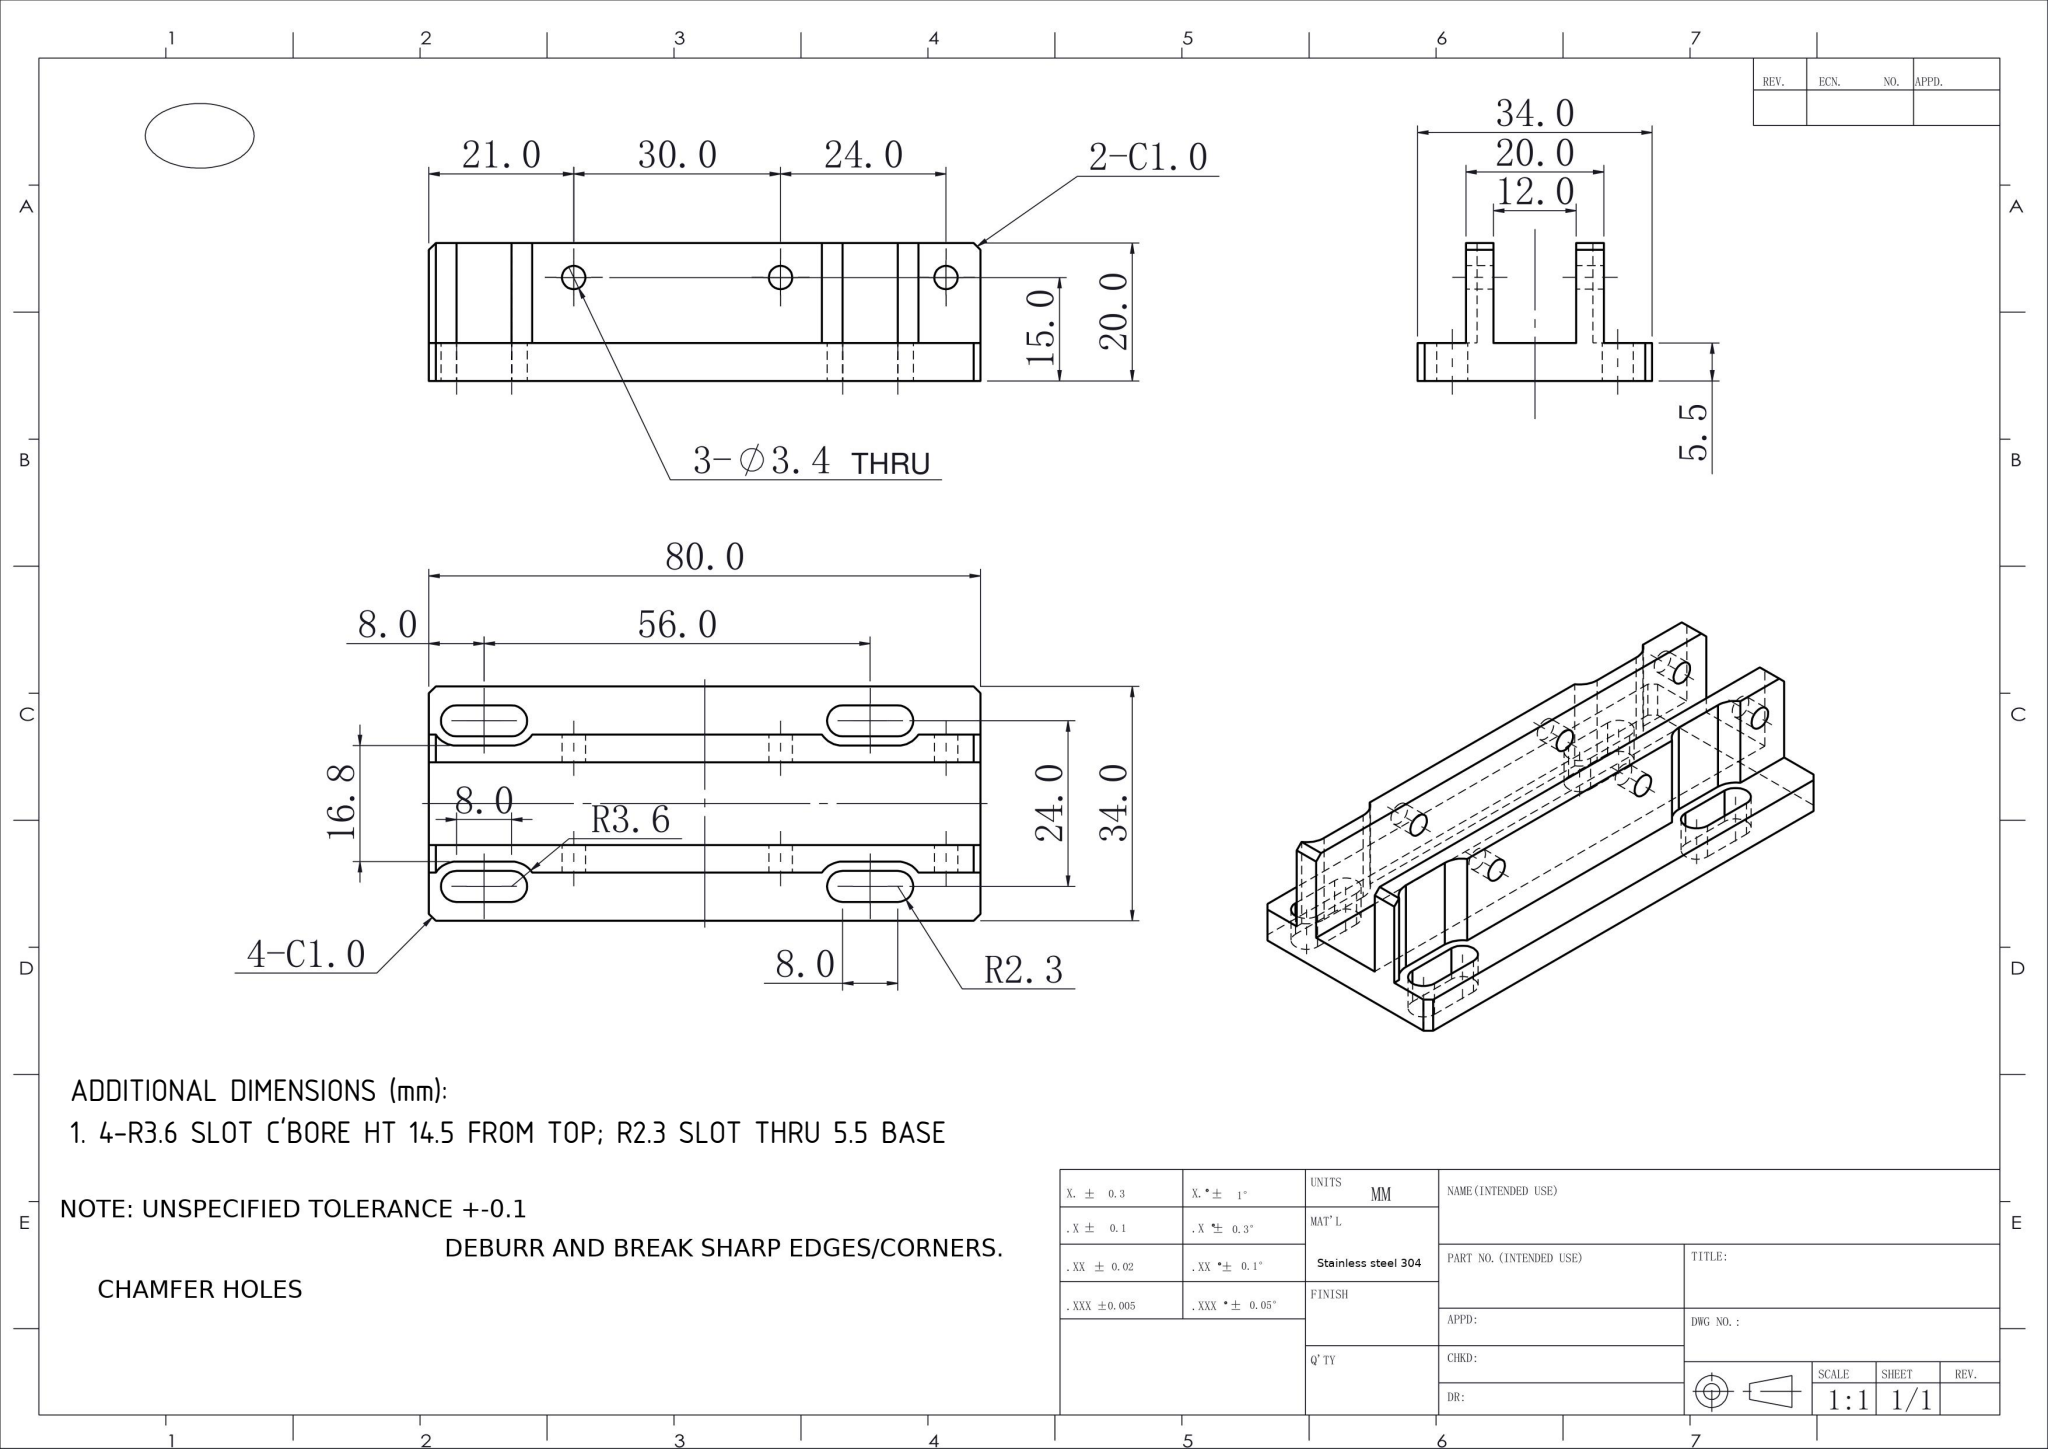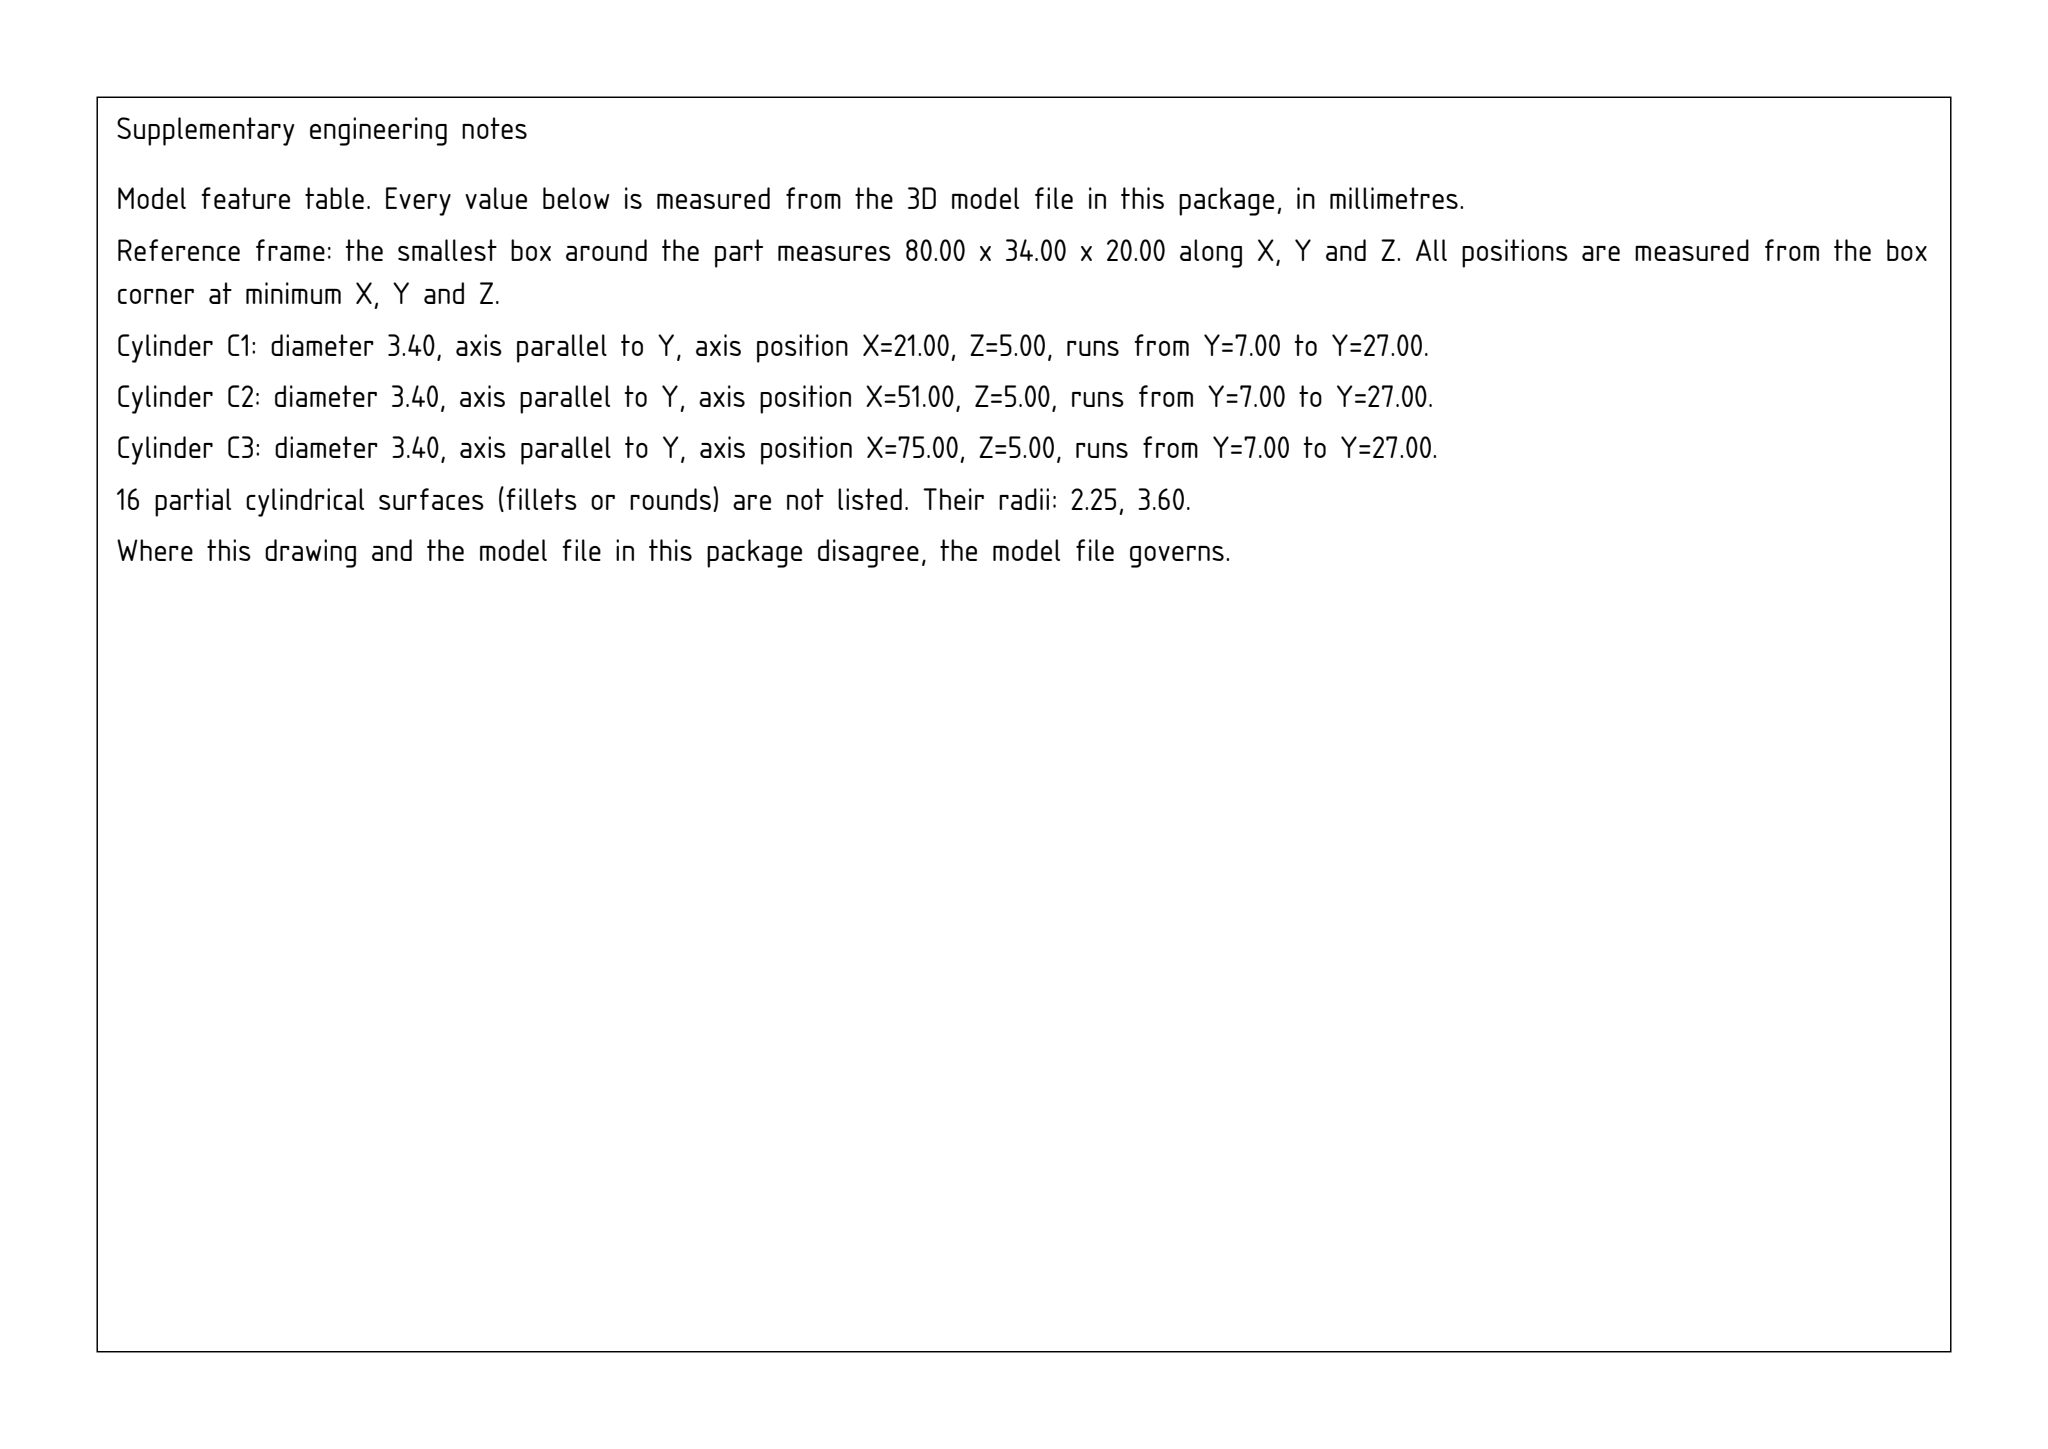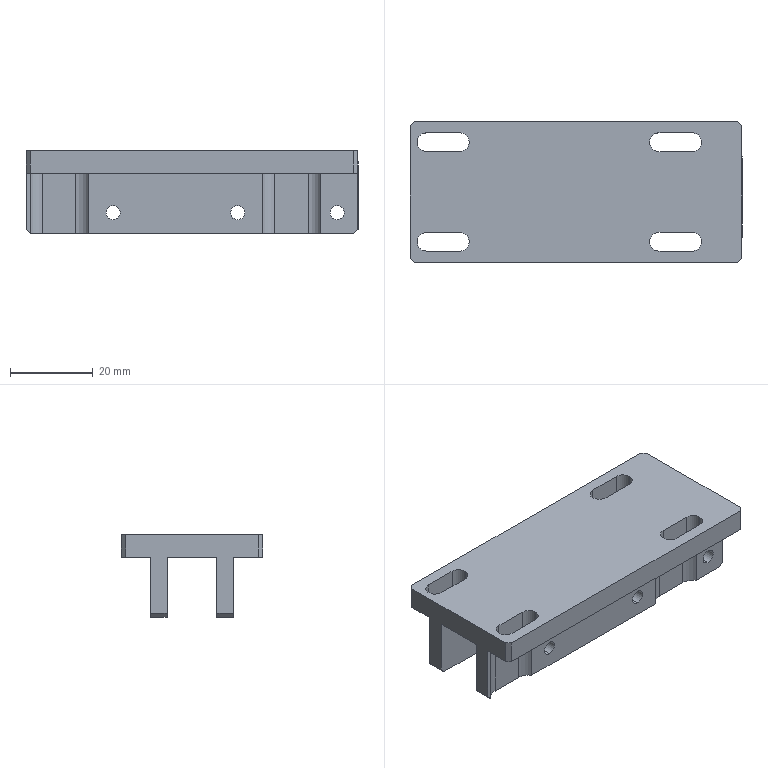Part | SolidWorks | mm | 1 solid | 70 faces | box 80 x 34 x 20 mm | volume 21728 mm3 | plane 38 | cylinder 32 | commonest cylinder face diameters 3.4 x12 4.5 x12 7.2 x8
build123d program:
from build123d import *

# Parameters (mm, degrees)
SKETCH1_W           = 80
SKETCH1_H           = 34
BOSS_EXTRUDE1_DEPTH = 20
SKETCH2_W           = 80
SKETCH2_H           = 12
CUT_EXTRUDE1_DEPTH  = 14.5
SKETCH5_W           = 80
SKETCH5_H           = 7
CUT_EXTRUDE2_DEPTH  = 46.818
CUT_EXTRUDE3_DEPTH  = 48.843
CUT_EXTRUDE4_DEPTH  = 46.818
CHAMFER1_SIZE       = 1
SKETCH10_R          = 1.7
CUT_EXTRUDE7_DEPTH  = 53.24
CHAMFER2_SIZE       = 1


with BuildPart() as part:
    # Sketch1 → Boss-Extrude1 (new body)
    with BuildSketch(Plane.XY):
        Rectangle(SKETCH1_W, SKETCH1_H)
    extrude(amount=-BOSS_EXTRUDE1_DEPTH)

    # Sketch2 → Cut-Extrude1 (cut)
    with BuildSketch(Plane(origin=(0, 0, -20), x_dir=(-1, 0, 0), z_dir=(0, 0, -1))):
        Rectangle(SKETCH2_W, SKETCH2_H)
    extrude(amount=-CUT_EXTRUDE1_DEPTH, mode=Mode.SUBTRACT)

    # Sketch5 → Cut-Extrude2 (cut, through all)
    with BuildSketch(Plane(origin=(0, 0, -5.5), x_dir=(-1, 0, 0), z_dir=(0, 0, -1))):
        with Locations((0, 13.5)):
            Rectangle(SKETCH5_W, SKETCH5_H)
        with Locations((0, -13.5)):
            Rectangle(SKETCH5_W, SKETCH5_H)
    extrude(amount=CUT_EXTRUDE2_DEPTH, mode=Mode.SUBTRACT)

    # Sketch6 → Cut-Extrude3 (cut, through all)
    with BuildSketch(Plane.XY):
        with BuildLine():
            Line((-36, 14.25), (-28, 14.25))
            ThreePointArc((-28, 14.25), (-25.75, 12), (-28, 9.75))
            Line((-28, 9.75), (-36, 9.75))
            ThreePointArc((-36, 9.75), (-38.25, 12), (-36, 14.25))
        make_face()
        with BuildLine():
            Line((20, 14.25), (28, 14.25))
            ThreePointArc((28, 14.25), (30.25, 12), (28, 9.75))
            Line((28, 9.75), (20, 9.75))
            ThreePointArc((20, 9.75), (17.75, 12), (20, 14.25))
        make_face()
        with BuildLine():
            Line((-36, -9.75), (-28, -9.75))
            ThreePointArc((-28, -9.75), (-25.75, -12), (-28, -14.25))
            Line((-28, -14.25), (-36, -14.25))
            ThreePointArc((-36, -14.25), (-38.25, -12), (-36, -9.75))
        make_face()
        with BuildLine():
            Line((20, -9.75), (28, -9.75))
            ThreePointArc((28, -9.75), (30.25, -12), (28, -14.25))
            Line((28, -14.25), (20, -14.25))
            ThreePointArc((20, -14.25), (17.75, -12), (20, -9.75))
        make_face()
    extrude(amount=-CUT_EXTRUDE3_DEPTH, mode=Mode.SUBTRACT)

    # Sketch7 → Cut-Extrude4 (cut, through all)
    with BuildSketch(Plane(origin=(0, 0, -5.5), x_dir=(-1, 0, 0), z_dir=(0, 0, -1))):
        with BuildLine():
            Line((-28, 15.6), (-20, 15.6))
            ThreePointArc((-20, 15.6), (-16.4, 12), (-20, 8.4))
            Line((-20, 8.4), (-28, 8.4))
            ThreePointArc((-28, 8.4), (-31.6, 12), (-28, 15.6))
        make_face()
        with BuildLine():
            Line((28, 15.6), (36, 15.6))
            ThreePointArc((36, 15.6), (39.6, 12), (36, 8.4))
            Line((36, 8.4), (28, 8.4))
            ThreePointArc((28, 8.4), (24.4, 12), (28, 15.6))
        make_face()
        with BuildLine():
            Line((36, -15.6), (28, -15.6))
            ThreePointArc((28, -15.6), (24.4, -12), (28, -8.4))
            Line((28, -8.4), (36, -8.4))
            ThreePointArc((36, -8.4), (39.6, -12), (36, -15.6))
        make_face()
        with BuildLine():
            Line((-20, -15.6), (-28, -15.6))
            ThreePointArc((-28, -15.6), (-31.6, -12), (-28, -8.4))
            Line((-28, -8.4), (-20, -8.4))
            ThreePointArc((-20, -8.4), (-16.4, -12), (-20, -15.6))
        make_face()
    extrude(amount=CUT_EXTRUDE4_DEPTH, mode=Mode.SUBTRACT)

    # Chamfer1
    chamfer1_edges = [part.edges().sort_by_distance(p)[0] for p in [
        (40, 17, -2.75),
        (-40, 17, -2.75),
        (-40, -17, -2.75),
        (40, -17, -2.75),
    ]]
    chamfer(chamfer1_edges, length=CHAMFER1_SIZE)

    # Sketch10 → Cut-Extrude7 (cut, through all)
    with BuildSketch(Plane.XZ.offset(10)):
        with Locations(Location((35, -15, 0), (0, 0, 90))):
            Circle(SKETCH10_R)
        with Locations(Location((11, -15, 0), (0, 0, 90))):
            Circle(SKETCH10_R)
        with Locations(Location((-19, -15, 0), (0, 0, 90))):
            Circle(SKETCH10_R)
    extrude(amount=-CUT_EXTRUDE7_DEPTH, mode=Mode.SUBTRACT)

    # Chamfer2
    chamfer2_edges = [part.edges().sort_by_distance(p)[0] for p in [
        (-40, -8, -20),
        (40, 8, -20),
        (-40, 8, -20),
        (40, -8, -20),
    ]]
    chamfer(chamfer2_edges, length=CHAMFER2_SIZE)


solid = part.part